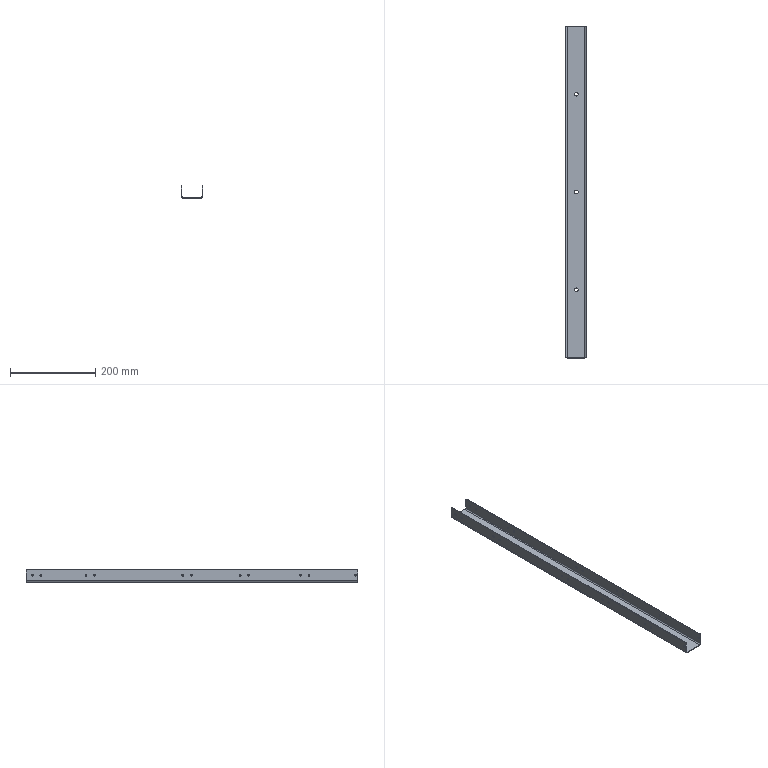Component | SolidWorks | FrameLongitudinalBeamFive100-2 | 1 solid | 76 faces | volume 121103 mm3 | cylinder 58 | plane 18 | commonest cylinder face diameters 4.5 x44 9 x6 6 x4 8 x2 5 x2